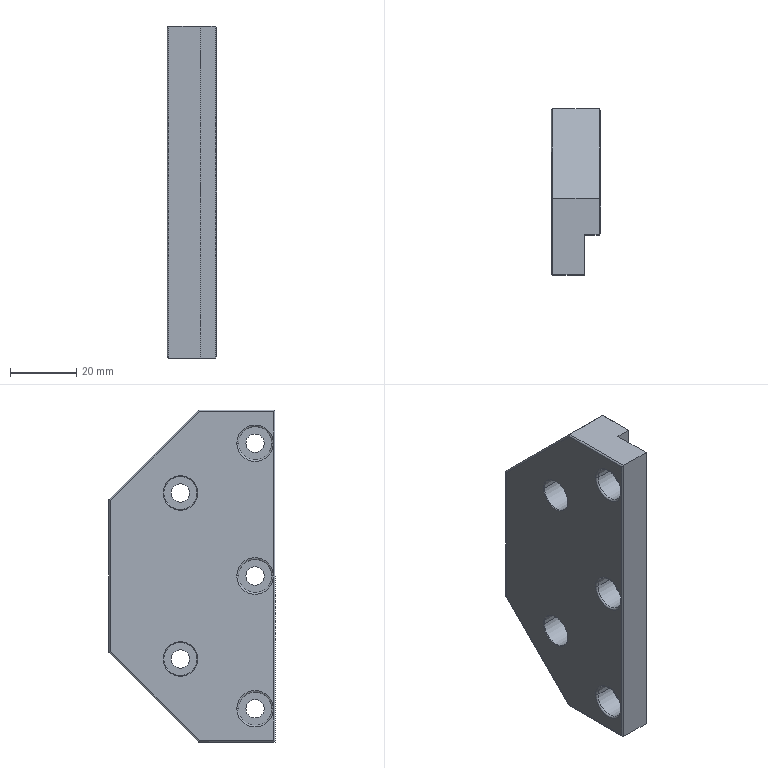Component | SolidWorks | Z-AxisElectricScrewdriverFixingPlateBottomPlate-1 | 1 solid | 67 faces | volume 54004 mm3 | cylinder 30 | plane 23 | cone 8 | torus 6 | commonest cylinder face diameters 10 x10 5.5 x10 1 x6 12.1 x4